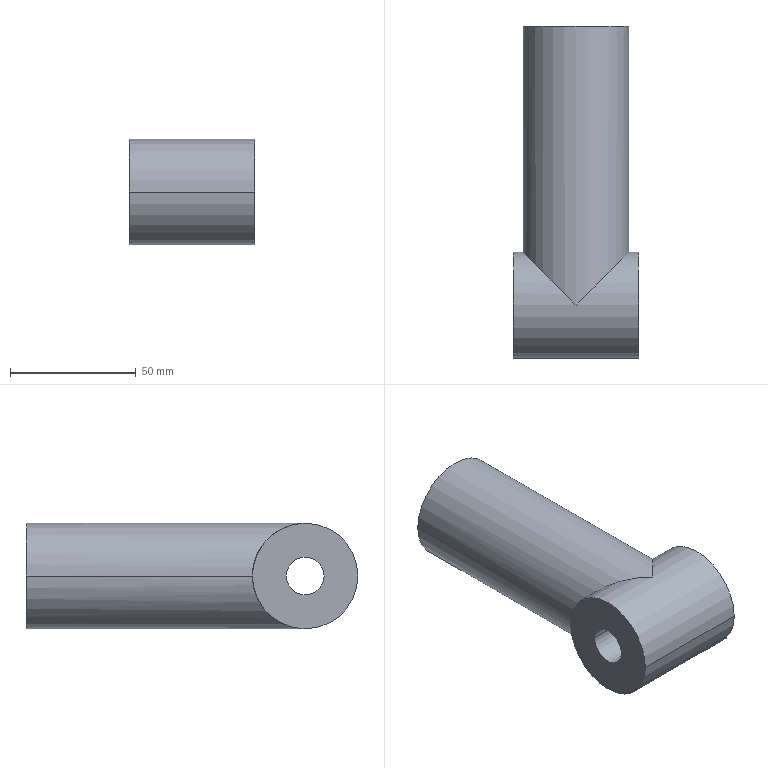Component | SolidWorks | CylinderAxis-2 | 1 solid | 9 faces | box 50 x 132 x 42 mm | volume 189524 mm3 | cylinder 6 | plane 3 | commonest cylinder face diameters 42 x4 15 x2
build123d program:
from build123d import *

# Parameters (mm, degrees)
SKETCH1_R                            = 21
SKETCH1_R_2                          = 7.5
BOSS_EXTRUDE1_DEPTH                  = 50
SKETCH2_R                            = 21
BOSS_EXTRUDE2_DEPTH                  = 90
BOSS_EXTRUDE2_DIRECTION_2_REACH      = 329.574
BOSS_EXTRUDE2_DIRECTION_2_END_RADIUS = 21


with BuildPart() as part:
    # Sketch1 → Boss-Extrude1 (new body)
    with BuildSketch(Plane.XY):
        with Locations((-120, 300)):
            Circle(SKETCH1_R)
        with Locations((-120, 300)):
            Circle(SKETCH1_R_2, mode=Mode.SUBTRACT)
    extrude(amount=BOSS_EXTRUDE1_DEPTH)

    # Sketch2 → Boss-Extrude2 (add)
    with BuildSketch(Plane(origin=(-99, 0, 0), x_dir=(0, 0, -1), z_dir=(1, 0, 0))):
        with Locations((-25, 300)):
            Circle(SKETCH2_R)
    extrude(amount=BOSS_EXTRUDE2_DEPTH)

    # Boss-Extrude2 direction 2: up to this cylinder (the profile starts outside it)
    boss_extrude2_direction_2_end = Plane(origin=(-120, 300, 25), z_dir=(0, 0, -1)) * Cylinder(BOSS_EXTRUDE2_DIRECTION_2_END_RADIUS, 702.148, mode=Mode.PRIVATE)
    # Sketch2 → Boss-Extrude2 direction 2 (add, up to the surface)
    with BuildSketch(Plane(origin=(-99, 0, 0), x_dir=(0, 0, -1), z_dir=(1, 0, 0)), mode=Mode.PRIVATE) as boss_extrude2_direction_2_sk1:
        with Locations((-25, 300)):
            Circle(SKETCH2_R)
    boss_extrude2_direction_2_tool1 = extrude(boss_extrude2_direction_2_sk1.sketch, amount=-BOSS_EXTRUDE2_DIRECTION_2_REACH, mode=Mode.PRIVATE) - boss_extrude2_direction_2_end
    add(boss_extrude2_direction_2_tool1.solids().sort_by_distance((-99, 300, 25))[0])
    add(boss_extrude2_direction_2_tool1.solids().sort_by_distance((-99, 300, 25))[1])


solid = part.part

# Placed as in the assembly
solid = solid.moved(Location((-250, -256, -600), (90, 90, 0)))
STEP:
#1=COLOUR_RGB('',0.7922,0.8196,0.9333);
#2=FILL_AREA_STYLE_COLOUR('',#1);
#3=FILL_AREA_STYLE('',(#2));
#4=SURFACE_STYLE_FILL_AREA(#3);
#5=SURFACE_SIDE_STYLE('',(#4));
#6=SURFACE_STYLE_USAGE(.BOTH.,#5);
#7=PRESENTATION_STYLE_ASSIGNMENT((#6));
#8=CARTESIAN_POINT('',(-8.031,-10.433,-11.811));
#9=VERTEX_POINT('',#8);
#10=CARTESIAN_POINT('',(-9.685,-10.433,-11.811));
#11=VERTEX_POINT('',#10);
#12=CARTESIAN_POINT('',(-8.858,-10.433,-11.811));
#13=DIRECTION('',(-0.,1.,0.));
#14=DIRECTION('',(1.,0.,0.));
#15=AXIS2_PLACEMENT_3D('',#12,#13,#14);
#16=CIRCLE('',#15,0.8268);
#17=EDGE_CURVE('',#9,#11,#16,.T.);
#18=ORIENTED_EDGE('',*,*,#17,.F.);
#19=CARTESIAN_POINT('',(-8.031,-13.976,-11.811));
#20=VERTEX_POINT('',#19);
#21=CARTESIAN_POINT('',(-8.031,-10.433,-11.811));
#22=DIRECTION('',(0.,-1.,-0.));
#23=VECTOR('',#22,39.37);
#24=LINE('',#21,#23);
#25=EDGE_CURVE('',#9,#20,#24,.T.);
#26=ORIENTED_EDGE('',*,*,#25,.T.);
#27=CARTESIAN_POINT('',(-8.858,-14.803,-12.638));
#28=VERTEX_POINT('',#27);
#29=CARTESIAN_POINT('',(-8.031,-13.976,-11.811));
#30=CARTESIAN_POINT('',(-8.031,-13.976,-12.295));
#31=CARTESIAN_POINT('',(-8.374,-14.319,-12.638));
#32=CARTESIAN_POINT('',(-8.858,-14.803,-12.638));
#33=(BOUNDED_CURVE()B_SPLINE_CURVE(3,(#29,#30,#31,#32),.UNSPECIFIED.,.F.,.F.)B_SPLINE_CURVE_WITH_KNOTS((4,4),(0.,1.571),.UNSPECIFIED.)CURVE()GEOMETRIC_REPRESENTATION_ITEM()RATIONAL_B_SPLINE_CURVE((1.,0.8047,0.8047,1.))REPRESENTATION_ITEM(''));
#34=EDGE_CURVE('',#20,#28,#33,.T.);
#35=ORIENTED_EDGE('',*,*,#34,.T.);
#36=CARTESIAN_POINT('',(-9.685,-13.976,-11.811));
#37=VERTEX_POINT('',#36);
#38=CARTESIAN_POINT('',(-8.858,-14.803,-12.638));
#39=CARTESIAN_POINT('',(-9.343,-14.319,-12.638));
#40=CARTESIAN_POINT('',(-9.685,-13.976,-12.295));
#41=CARTESIAN_POINT('',(-9.685,-13.976,-11.811));
#42=(BOUNDED_CURVE()B_SPLINE_CURVE(3,(#38,#39,#40,#41),.UNSPECIFIED.,.F.,.T.)B_SPLINE_CURVE_WITH_KNOTS((4,4),(4.712,6.283),.UNSPECIFIED.)CURVE()GEOMETRIC_REPRESENTATION_ITEM()RATIONAL_B_SPLINE_CURVE((1.,0.8047,0.8047,1.))REPRESENTATION_ITEM(''));
#43=EDGE_CURVE('',#28,#37,#42,.T.);
#44=ORIENTED_EDGE('',*,*,#43,.T.);
#45=CARTESIAN_POINT('',(-9.685,-10.433,-11.811));
#46=DIRECTION('',(0.,-1.,-0.));
#47=VECTOR('',#46,39.37);
#48=LINE('',#45,#47);
#49=EDGE_CURVE('',#11,#37,#48,.T.);
#50=ORIENTED_EDGE('',*,*,#49,.F.);
#51=EDGE_LOOP('',(#18,#26,#35,#44,#50));
#52=FACE_OUTER_BOUND('',#51,.T.);
#53=CARTESIAN_POINT('',(-8.858,-10.433,-11.811));
#54=DIRECTION('',(0.,-1.,-0.));
#55=DIRECTION('',(-1.,0.,0.));
#56=AXIS2_PLACEMENT_3D('',#53,#54,#55);
#57=CYLINDRICAL_SURFACE('',#56,0.8268);
#58=ADVANCED_FACE('',(#52),#57,.T.);
#59=CARTESIAN_POINT('',(-9.843,-15.098,-11.811));
#60=VERTEX_POINT('',#59);
#61=CARTESIAN_POINT('',(-9.843,-14.508,-11.811));
#62=VERTEX_POINT('',#61);
#63=CARTESIAN_POINT('',(-9.843,-14.803,-11.811));
#64=DIRECTION('',(-1.,-0.,-0.));
#65=DIRECTION('',(0.,1.,0.));
#66=AXIS2_PLACEMENT_3D('',#63,#64,#65);
#67=CIRCLE('',#66,0.2953);
#68=EDGE_CURVE('',#60,#62,#67,.T.);
#69=ORIENTED_EDGE('',*,*,#68,.T.);
#70=CARTESIAN_POINT('',(-7.874,-14.508,-11.811));
#71=VERTEX_POINT('',#70);
#72=CARTESIAN_POINT('',(-9.843,-14.508,-11.811));
#73=DIRECTION('',(1.,0.,0.));
#74=VECTOR('',#73,39.37);
#75=LINE('',#72,#74);
#76=EDGE_CURVE('',#62,#71,#75,.T.);
#77=ORIENTED_EDGE('',*,*,#76,.T.);
#78=CARTESIAN_POINT('',(-7.874,-15.098,-11.811));
#79=VERTEX_POINT('',#78);
#80=CARTESIAN_POINT('',(-7.874,-14.803,-11.811));
#81=DIRECTION('',(-1.,-0.,-0.));
#82=DIRECTION('',(0.,1.,0.));
#83=AXIS2_PLACEMENT_3D('',#80,#81,#82);
#84=CIRCLE('',#83,0.2953);
#85=EDGE_CURVE('',#79,#71,#84,.T.);
#86=ORIENTED_EDGE('',*,*,#85,.F.);
#87=CARTESIAN_POINT('',(-9.843,-15.098,-11.811));
#88=DIRECTION('',(1.,0.,0.));
#89=VECTOR('',#88,39.37);
#90=LINE('',#87,#89);
#91=EDGE_CURVE('',#60,#79,#90,.T.);
#92=ORIENTED_EDGE('',*,*,#91,.F.);
#93=EDGE_LOOP('',(#69,#77,#86,#92));
#94=FACE_OUTER_BOUND('',#93,.T.);
#95=CARTESIAN_POINT('',(-9.843,-14.803,-11.811));
#96=DIRECTION('',(1.,0.,0.));
#97=DIRECTION('',(0.,-1.,0.));
#98=AXIS2_PLACEMENT_3D('',#95,#96,#97);
#99=CYLINDRICAL_SURFACE('',#98,0.2953);
#100=ADVANCED_FACE('',(#94),#99,.F.);
#101=CARTESIAN_POINT('',(-9.843,-13.976,-11.811));
#102=VERTEX_POINT('',#101);
#103=CARTESIAN_POINT('',(-9.843,-15.63,-11.811));
#104=VERTEX_POINT('',#103);
#105=CARTESIAN_POINT('',(-9.843,-14.803,-11.811));
#106=DIRECTION('',(-1.,-0.,-0.));
#107=DIRECTION('',(0.,1.,0.));
#108=AXIS2_PLACEMENT_3D('',#105,#106,#107);
#109=CIRCLE('',#108,0.8268);
#110=EDGE_CURVE('',#102,#104,#109,.T.);
#111=ORIENTED_EDGE('',*,*,#110,.F.);
#112=CARTESIAN_POINT('',(-9.843,-13.976,-11.811));
#113=DIRECTION('',(1.,0.,0.));
#114=VECTOR('',#113,39.37);
#115=LINE('',#112,#114);
#116=EDGE_CURVE('',#102,#37,#115,.T.);
#117=ORIENTED_EDGE('',*,*,#116,.T.);
#118=ORIENTED_EDGE('',*,*,#43,.F.);
#119=ORIENTED_EDGE('',*,*,#34,.F.);
#120=CARTESIAN_POINT('',(-7.874,-13.976,-11.811));
#121=VERTEX_POINT('',#120);
#122=CARTESIAN_POINT('',(-9.843,-13.976,-11.811));
#123=DIRECTION('',(1.,0.,0.));
#124=VECTOR('',#123,39.37);
#125=LINE('',#122,#124);
#126=EDGE_CURVE('',#20,#121,#125,.T.);
#127=ORIENTED_EDGE('',*,*,#126,.T.);
#128=CARTESIAN_POINT('',(-7.874,-15.63,-11.811));
#129=VERTEX_POINT('',#128);
#130=CARTESIAN_POINT('',(-7.874,-14.803,-11.811));
#131=DIRECTION('',(-1.,-0.,-0.));
#132=DIRECTION('',(0.,1.,0.));
#133=AXIS2_PLACEMENT_3D('',#130,#131,#132);
#134=CIRCLE('',#133,0.8268);
#135=EDGE_CURVE('',#121,#129,#134,.T.);
#136=ORIENTED_EDGE('',*,*,#135,.T.);
#137=CARTESIAN_POINT('',(-9.843,-15.63,-11.811));
#138=DIRECTION('',(1.,0.,0.));
#139=VECTOR('',#138,39.37);
#140=LINE('',#137,#139);
#141=EDGE_CURVE('',#104,#129,#140,.T.);
#142=ORIENTED_EDGE('',*,*,#141,.F.);
#143=EDGE_LOOP('',(#111,#117,#118,#119,#127,#136,#142));
#144=FACE_OUTER_BOUND('',#143,.T.);
#145=CARTESIAN_POINT('',(-9.843,-14.803,-11.811));
#146=DIRECTION('',(1.,0.,0.));
#147=DIRECTION('',(0.,-1.,0.));
#148=AXIS2_PLACEMENT_3D('',#145,#146,#147);
#149=CYLINDRICAL_SURFACE('',#148,0.8268);
#150=ADVANCED_FACE('',(#144),#149,.T.);
#151=ORIENTED_EDGE('',*,*,#116,.F.);
#152=CARTESIAN_POINT('',(-9.843,-14.803,-11.811));
#153=DIRECTION('',(-1.,-0.,-0.));
#154=DIRECTION('',(0.,1.,0.));
#155=AXIS2_PLACEMENT_3D('',#152,#153,#154);
#156=CIRCLE('',#155,0.8268);
#157=EDGE_CURVE('',#104,#102,#156,.T.);
#158=ORIENTED_EDGE('',*,*,#157,.F.);
#159=ORIENTED_EDGE('',*,*,#141,.T.);
#160=CARTESIAN_POINT('',(-7.874,-14.803,-11.811));
#161=DIRECTION('',(-1.,-0.,-0.));
#162=DIRECTION('',(0.,1.,0.));
#163=AXIS2_PLACEMENT_3D('',#160,#161,#162);
#164=CIRCLE('',#163,0.8268);
#165=EDGE_CURVE('',#129,#121,#164,.T.);
#166=ORIENTED_EDGE('',*,*,#165,.T.);
#167=ORIENTED_EDGE('',*,*,#126,.F.);
#168=CARTESIAN_POINT('',(-8.858,-14.803,-10.984));
#169=VERTEX_POINT('',#168);
#170=CARTESIAN_POINT('',(-8.858,-14.803,-10.984));
#171=CARTESIAN_POINT('',(-8.374,-14.319,-10.984));
#172=CARTESIAN_POINT('',(-8.031,-13.976,-11.327));
#173=CARTESIAN_POINT('',(-8.031,-13.976,-11.811));
#174=(BOUNDED_CURVE()B_SPLINE_CURVE(3,(#170,#171,#172,#173),.UNSPECIFIED.,.F.,.F.)B_SPLINE_CURVE_WITH_KNOTS((4,4),(4.712,6.283),.UNSPECIFIED.)CURVE()GEOMETRIC_REPRESENTATION_ITEM()RATIONAL_B_SPLINE_CURVE((1.,0.8047,0.8047,1.))REPRESENTATION_ITEM(''));
#175=EDGE_CURVE('',#169,#20,#174,.T.);
#176=ORIENTED_EDGE('',*,*,#175,.F.);
#177=CARTESIAN_POINT('',(-9.685,-13.976,-11.811));
#178=CARTESIAN_POINT('',(-9.685,-13.976,-11.327));
#179=CARTESIAN_POINT('',(-9.343,-14.319,-10.984));
#180=CARTESIAN_POINT('',(-8.858,-14.803,-10.984));
#181=(BOUNDED_CURVE()B_SPLINE_CURVE(3,(#177,#178,#179,#180),.UNSPECIFIED.,.F.,.T.)B_SPLINE_CURVE_WITH_KNOTS((4,4),(-0.,1.571),.UNSPECIFIED.)CURVE()GEOMETRIC_REPRESENTATION_ITEM()RATIONAL_B_SPLINE_CURVE((1.,0.8047,0.8047,1.))REPRESENTATION_ITEM(''));
#182=EDGE_CURVE('',#37,#169,#181,.T.);
#183=ORIENTED_EDGE('',*,*,#182,.F.);
#184=EDGE_LOOP('',(#151,#158,#159,#166,#167,#176,#183));
#185=FACE_OUTER_BOUND('',#184,.T.);
#186=CARTESIAN_POINT('',(-9.843,-14.803,-11.811));
#187=DIRECTION('',(1.,0.,0.));
#188=DIRECTION('',(0.,-1.,0.));
#189=AXIS2_PLACEMENT_3D('',#186,#187,#188);
#190=CYLINDRICAL_SURFACE('',#189,0.8268);
#191=ADVANCED_FACE('',(#185),#190,.T.);
#192=ORIENTED_EDGE('',*,*,#157,.T.);
#193=ORIENTED_EDGE('',*,*,#110,.T.);
#194=EDGE_LOOP('',(#192,#193));
#195=FACE_OUTER_BOUND('',#194,.T.);
#196=ORIENTED_EDGE('',*,*,#68,.F.);
#197=CARTESIAN_POINT('',(-9.843,-14.803,-11.811));
#198=DIRECTION('',(-1.,-0.,-0.));
#199=DIRECTION('',(0.,1.,0.));
#200=AXIS2_PLACEMENT_3D('',#197,#198,#199);
#201=CIRCLE('',#200,0.2953);
#202=EDGE_CURVE('',#62,#60,#201,.T.);
#203=ORIENTED_EDGE('',*,*,#202,.F.);
#204=EDGE_LOOP('',(#196,#203));
#205=FACE_BOUND('',#204,.T.);
#206=CARTESIAN_POINT('',(-9.843,-14.803,-11.811));
#207=DIRECTION('',(-1.,-0.,-0.));
#208=DIRECTION('',(-0.,1.,0.));
#209=AXIS2_PLACEMENT_3D('',#206,#207,#208);
#210=PLANE('',#209);
#211=ADVANCED_FACE('',(#195,#205),#210,.T.);
#212=ORIENTED_EDGE('',*,*,#165,.F.);
#213=ORIENTED_EDGE('',*,*,#135,.F.);
#214=EDGE_LOOP('',(#212,#213));
#215=FACE_OUTER_BOUND('',#214,.T.);
#216=ORIENTED_EDGE('',*,*,#85,.T.);
#217=CARTESIAN_POINT('',(-7.874,-14.803,-11.811));
#218=DIRECTION('',(-1.,-0.,-0.));
#219=DIRECTION('',(0.,1.,0.));
#220=AXIS2_PLACEMENT_3D('',#217,#218,#219);
#221=CIRCLE('',#220,0.2953);
#222=EDGE_CURVE('',#71,#79,#221,.T.);
#223=ORIENTED_EDGE('',*,*,#222,.T.);
#224=EDGE_LOOP('',(#216,#223));
#225=FACE_BOUND('',#224,.T.);
#226=CARTESIAN_POINT('',(-7.874,-14.803,-11.811));
#227=DIRECTION('',(-1.,-0.,-0.));
#228=DIRECTION('',(-0.,1.,0.));
#229=AXIS2_PLACEMENT_3D('',#226,#227,#228);
#230=PLANE('',#229);
#231=ADVANCED_FACE('',(#215,#225),#230,.F.);
#232=ORIENTED_EDGE('',*,*,#76,.F.);
#233=ORIENTED_EDGE('',*,*,#202,.T.);
#234=ORIENTED_EDGE('',*,*,#91,.T.);
#235=ORIENTED_EDGE('',*,*,#222,.F.);
#236=EDGE_LOOP('',(#232,#233,#234,#235));
#237=FACE_OUTER_BOUND('',#236,.T.);
#238=CARTESIAN_POINT('',(-9.843,-14.803,-11.811));
#239=DIRECTION('',(1.,0.,0.));
#240=DIRECTION('',(0.,-1.,0.));
#241=AXIS2_PLACEMENT_3D('',#238,#239,#240);
#242=CYLINDRICAL_SURFACE('',#241,0.2953);
#243=ADVANCED_FACE('',(#237),#242,.F.);
#244=ORIENTED_EDGE('',*,*,#25,.F.);
#245=CARTESIAN_POINT('',(-8.858,-10.433,-11.811));
#246=DIRECTION('',(-0.,1.,0.));
#247=DIRECTION('',(1.,0.,0.));
#248=AXIS2_PLACEMENT_3D('',#245,#246,#247);
#249=CIRCLE('',#248,0.8268);
#250=EDGE_CURVE('',#11,#9,#249,.T.);
#251=ORIENTED_EDGE('',*,*,#250,.F.);
#252=ORIENTED_EDGE('',*,*,#49,.T.);
#253=ORIENTED_EDGE('',*,*,#182,.T.);
#254=ORIENTED_EDGE('',*,*,#175,.T.);
#255=EDGE_LOOP('',(#244,#251,#252,#253,#254));
#256=FACE_OUTER_BOUND('',#255,.T.);
#257=CARTESIAN_POINT('',(-8.858,-10.433,-11.811));
#258=DIRECTION('',(0.,-1.,-0.));
#259=DIRECTION('',(-1.,0.,0.));
#260=AXIS2_PLACEMENT_3D('',#257,#258,#259);
#261=CYLINDRICAL_SURFACE('',#260,0.8268);
#262=ADVANCED_FACE('',(#256),#261,.T.);
#263=ORIENTED_EDGE('',*,*,#250,.T.);
#264=ORIENTED_EDGE('',*,*,#17,.T.);
#265=EDGE_LOOP('',(#263,#264));
#266=FACE_OUTER_BOUND('',#265,.T.);
#267=CARTESIAN_POINT('',(-8.858,-10.433,-11.811));
#268=DIRECTION('',(-0.,1.,0.));
#269=DIRECTION('',(1.,0.,0.));
#270=AXIS2_PLACEMENT_3D('',#267,#268,#269);
#271=PLANE('',#270);
#272=ADVANCED_FACE('',(#266),#271,.T.);
#273=CLOSED_SHELL('',(#58,#100,#150,#191,#211,#231,#243,#262,#272));
#274=MANIFOLD_SOLID_BREP('',#273);
#275=STYLED_ITEM('',(#7),#274);
#276=PRESENTATION_LAYER_ASSIGNMENT('','',(#275));
#277=(LENGTH_UNIT()NAMED_UNIT(*)SI_UNIT($,.METRE.));
#278=LENGTH_MEASURE_WITH_UNIT(LENGTH_MEASURE(0.0254),#277);
#279=DIMENSIONAL_EXPONENTS(1.,0.,0.,0.,0.,0.,0.);
#280=(CONVERSION_BASED_UNIT('',#278)LENGTH_UNIT()NAMED_UNIT(#279));
#281=UNCERTAINTY_MEASURE_WITH_UNIT(LENGTH_MEASURE(0.00001),#280,'','');
#282=(NAMED_UNIT(*)PLANE_ANGLE_UNIT()SI_UNIT($,.RADIAN.));
#283=(NAMED_UNIT(*)SI_UNIT($,.STERADIAN.)SOLID_ANGLE_UNIT());
#284=(GEOMETRIC_REPRESENTATION_CONTEXT(3)GLOBAL_UNCERTAINTY_ASSIGNED_CONTEXT((#281))GLOBAL_UNIT_ASSIGNED_CONTEXT((#280,#282,#283))REPRESENTATION_CONTEXT('',''));
#285=MECHANICAL_DESIGN_GEOMETRIC_PRESENTATION_REPRESENTATION('',(#275),#284);
#286=CARTESIAN_POINT('',(0.,0.,0.));
#287=DIRECTION('',(0.,0.,1.));
#288=DIRECTION('',(1.,0.,0.));
#289=AXIS2_PLACEMENT_3D('',#286,#287,#288);
#290=(LENGTH_UNIT()NAMED_UNIT(*)SI_UNIT($,.METRE.));
#291=LENGTH_MEASURE_WITH_UNIT(LENGTH_MEASURE(0.0254),#290);
#292=DIMENSIONAL_EXPONENTS(1.,0.,0.,0.,0.,0.,0.);
#293=(CONVERSION_BASED_UNIT('',#291)LENGTH_UNIT()NAMED_UNIT(#292));
#294=UNCERTAINTY_MEASURE_WITH_UNIT(LENGTH_MEASURE(0.00001),#293,'','');
#295=(NAMED_UNIT(*)PLANE_ANGLE_UNIT()SI_UNIT($,.RADIAN.));
#296=(NAMED_UNIT(*)SI_UNIT($,.STERADIAN.)SOLID_ANGLE_UNIT());
#297=(GEOMETRIC_REPRESENTATION_CONTEXT(3)GLOBAL_UNCERTAINTY_ASSIGNED_CONTEXT((#294))GLOBAL_UNIT_ASSIGNED_CONTEXT((#293,#295,#296))REPRESENTATION_CONTEXT('',''));
#298=ADVANCED_BREP_SHAPE_REPRESENTATION('',(#274,#289),#297);